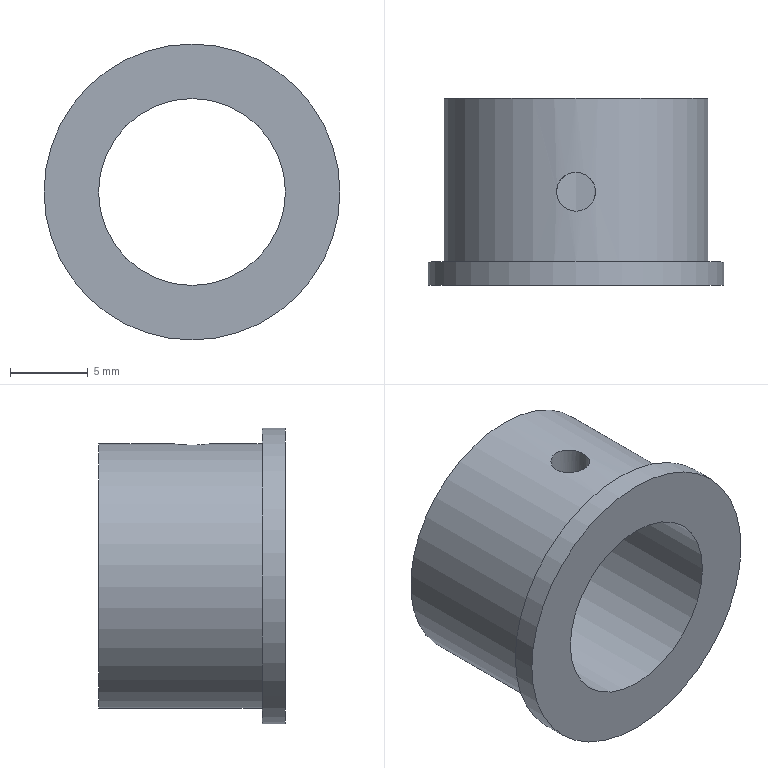Component | NX | PEDESTAL_BEARING_2 | 1 solid | 7 faces | volume 1439 mm3 | cylinder 4 | plane 3 | commonest cylinder face diameters 17 x1 12 x1 19 x1 2.5 x1